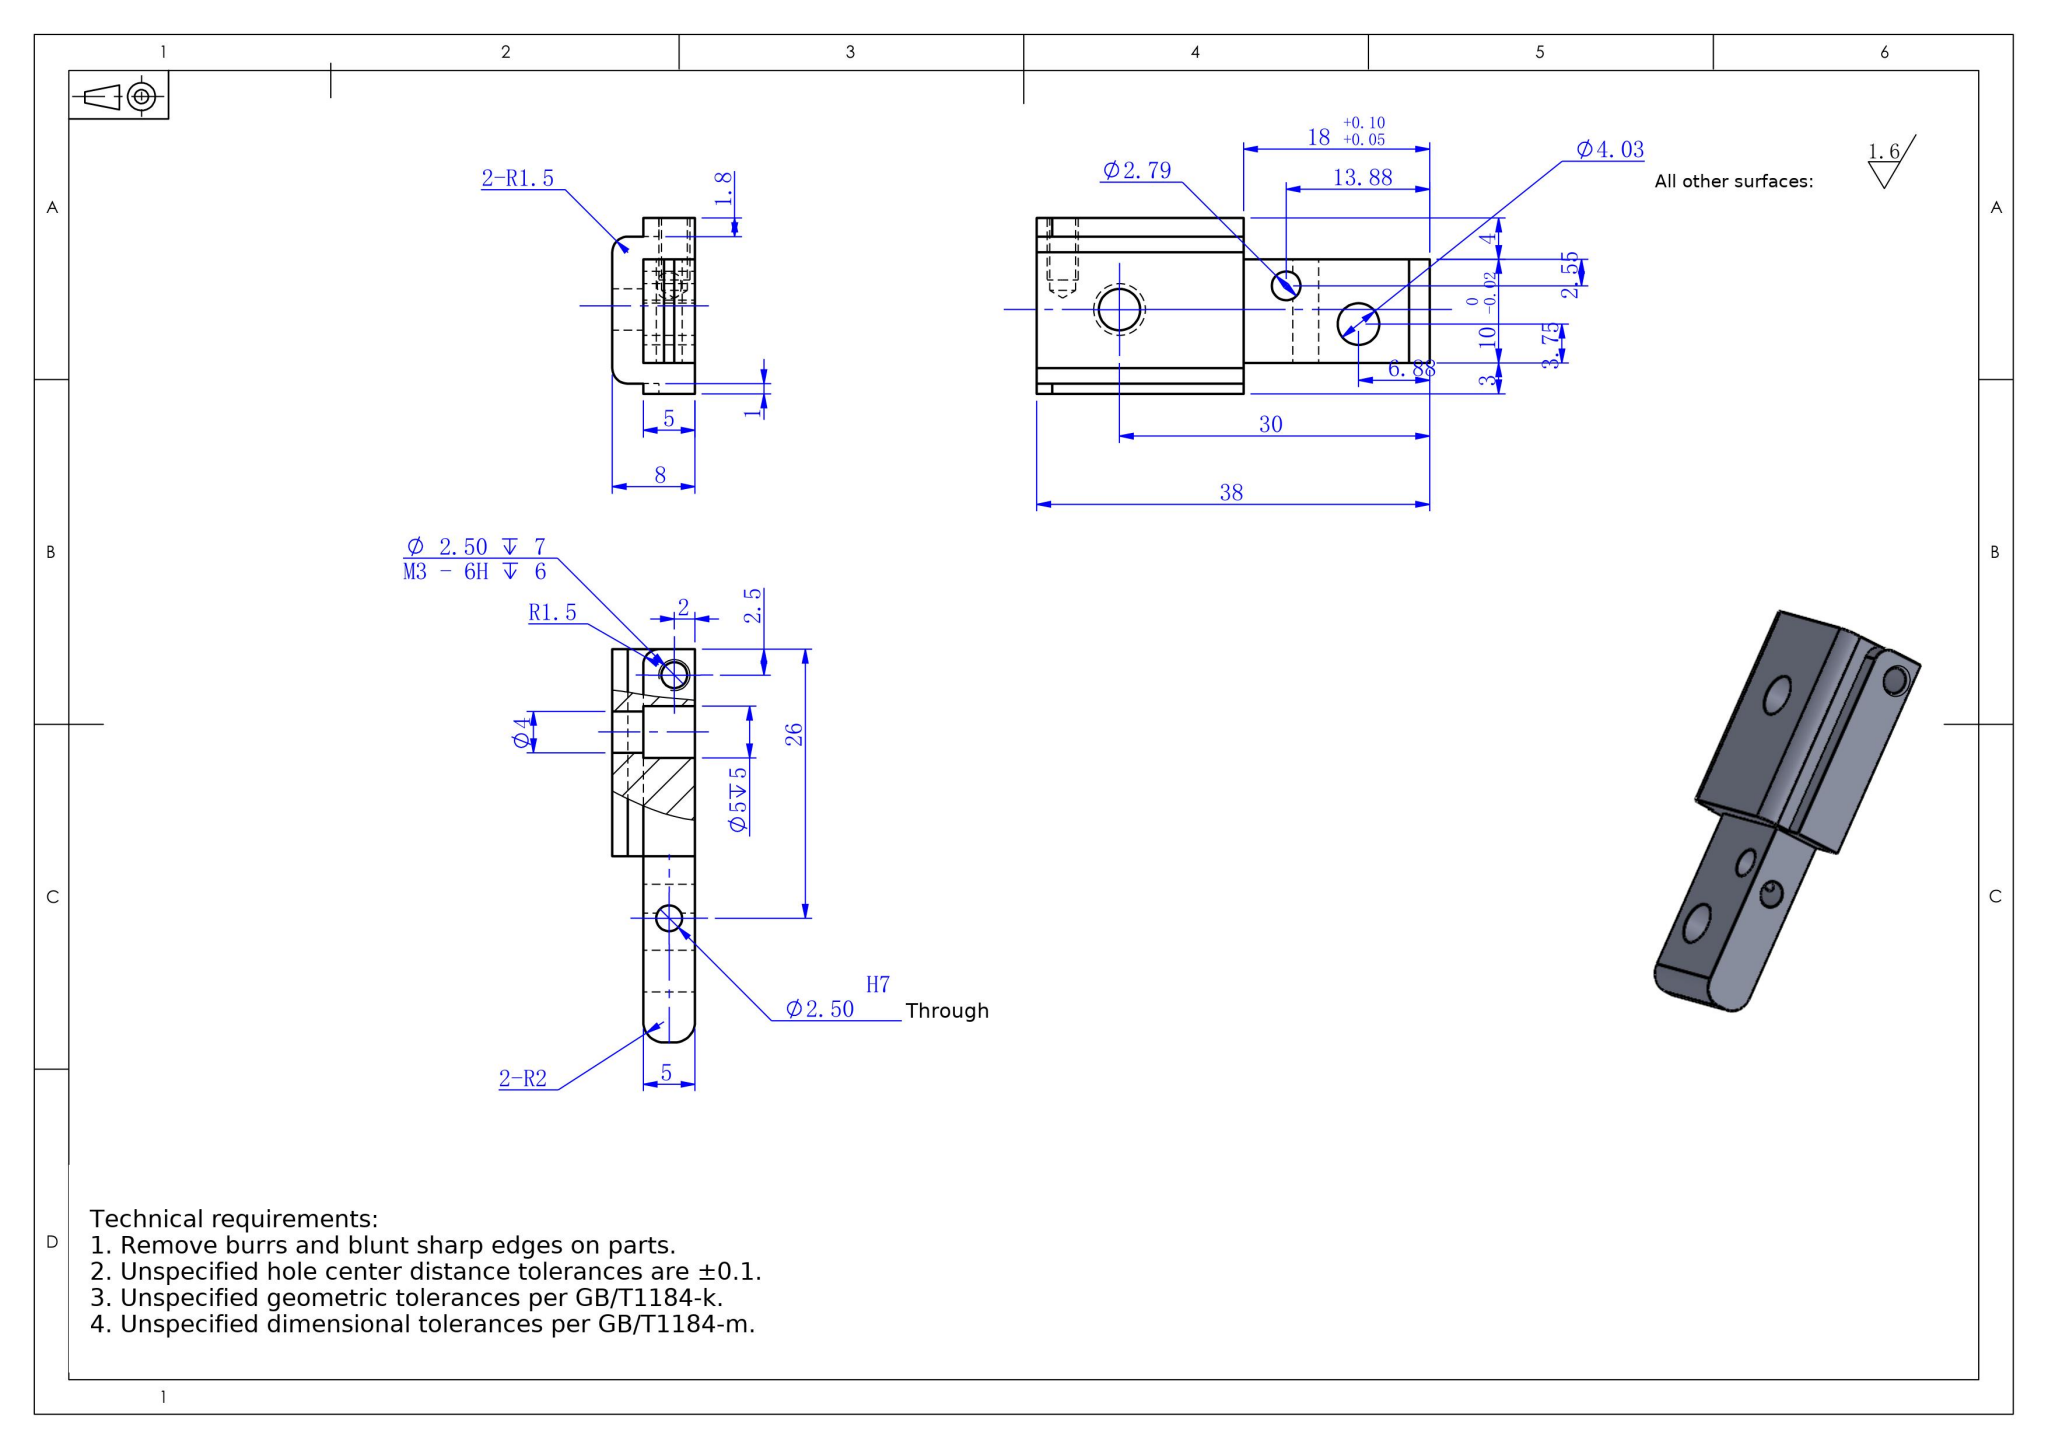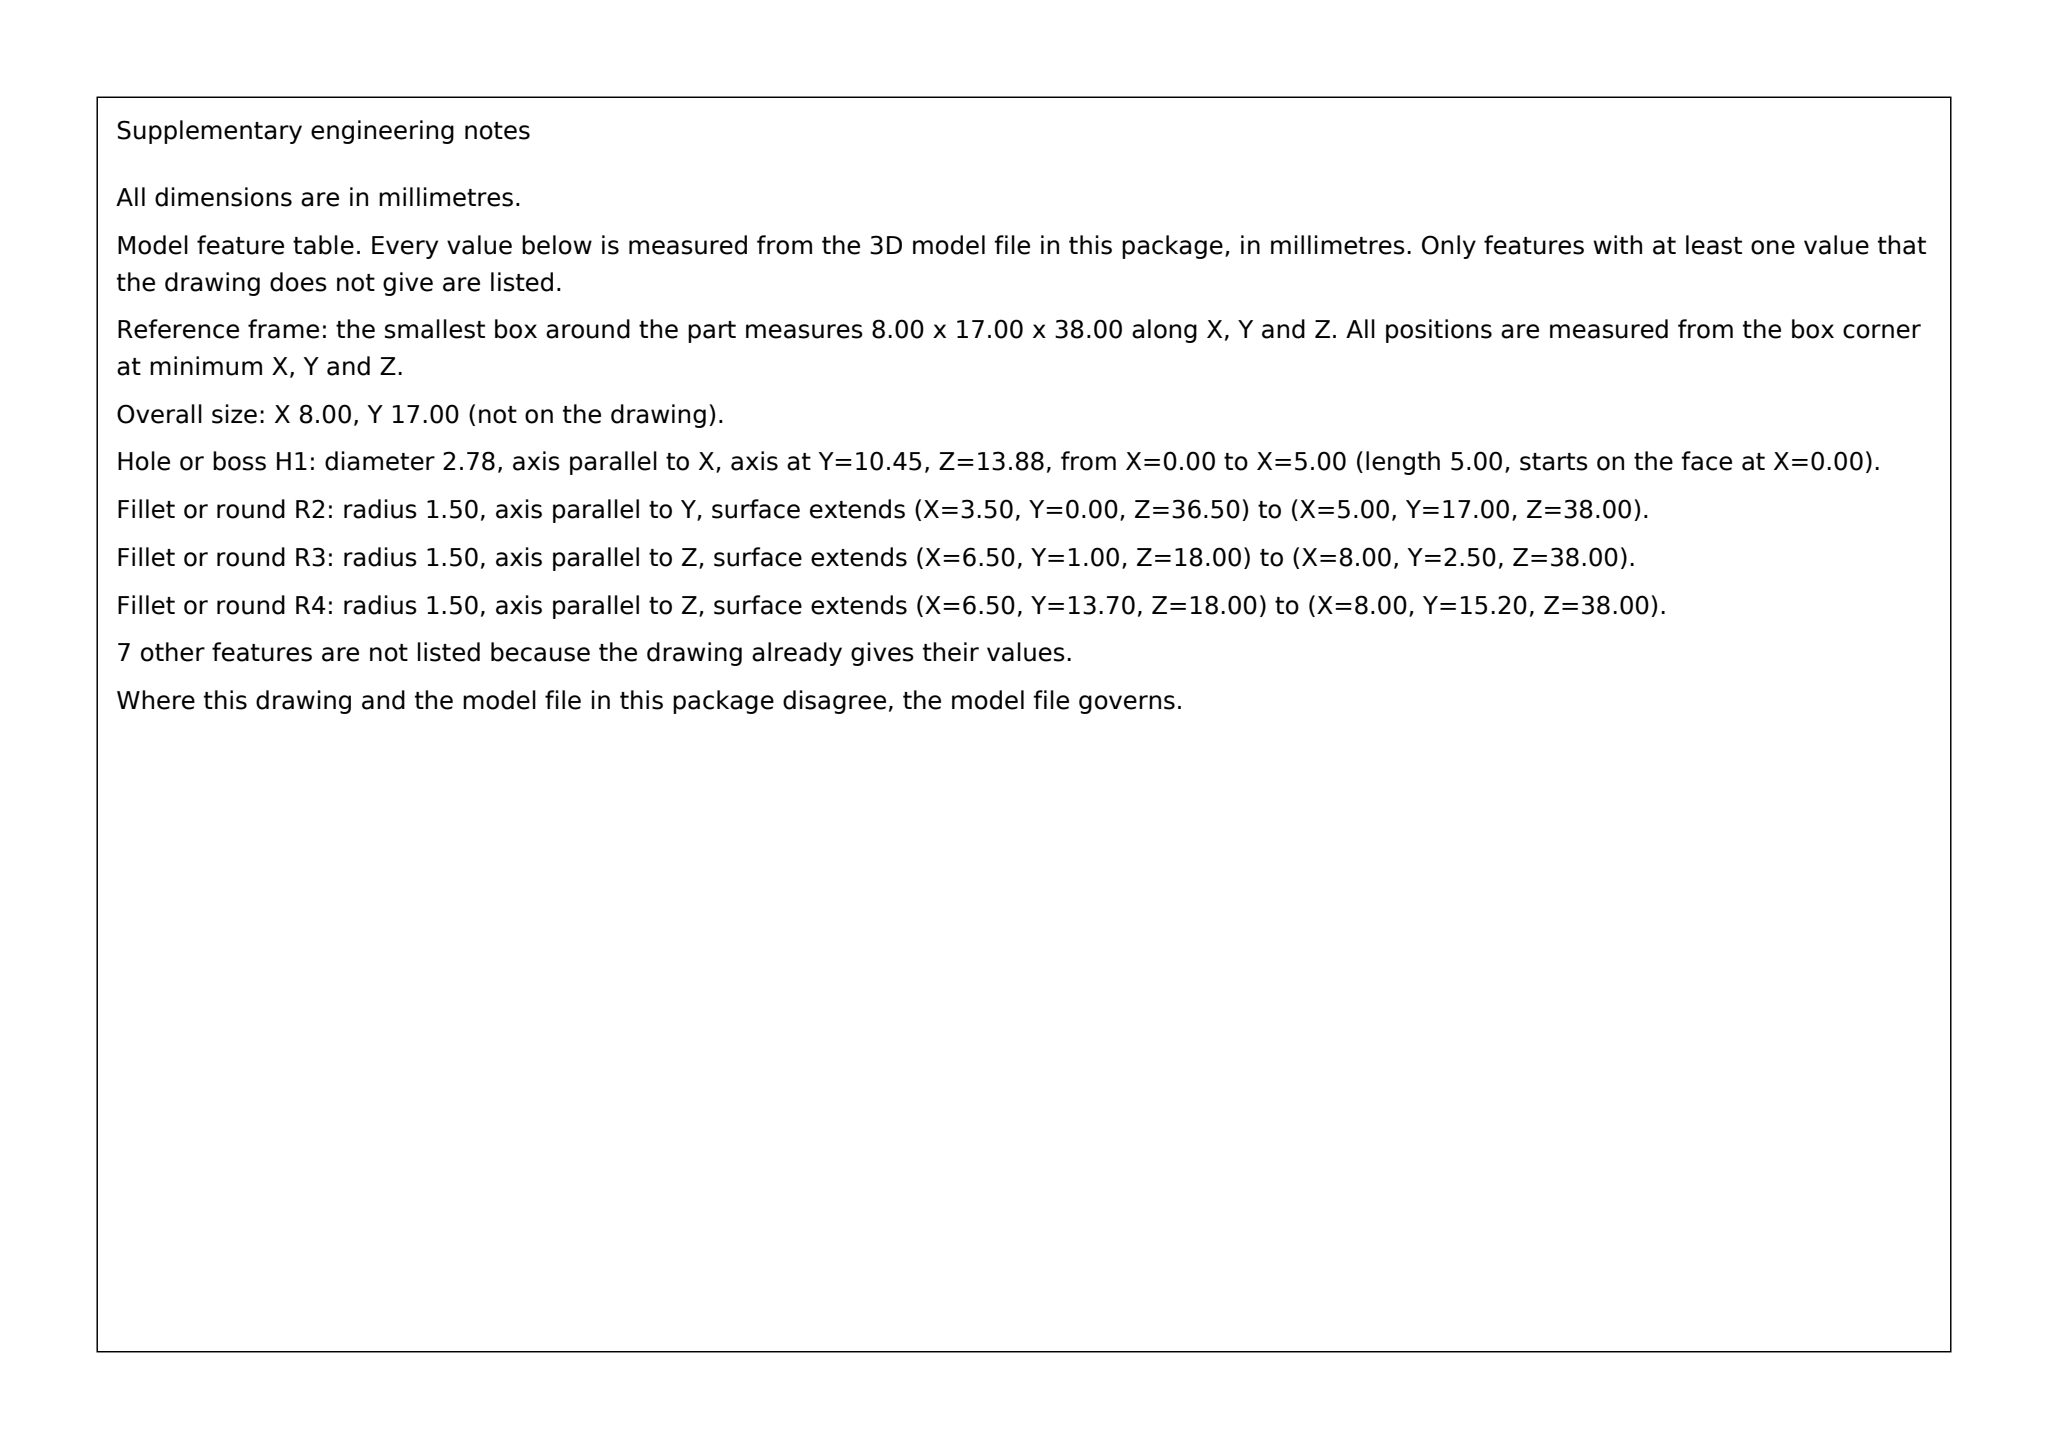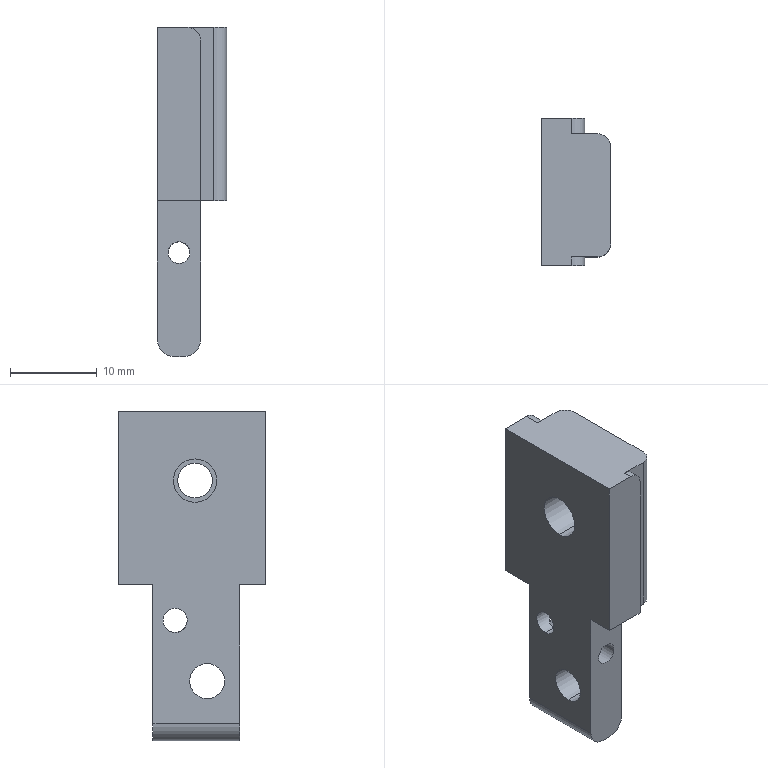Part | SolidWorks | mm | 1 solid | 35 faces | box 8 x 17 x 38 mm | volume 3101 mm3 | cylinder 18 | plane 15 | cone 2 | commonest cylinder face diameters 4 x4 2.5 x4 3 x4 4.029 x2 2.79 x2 5 x2
build123d program:
from build123d import *

# Parameters (mm, degrees)
SKETCH1_W             = 5
SKETCH1_H             = 17
BOSS_EXTRUDE1_DEPTH   = 20
SKETCH2_W             = 5
SKETCH2_H             = 10
BOSS_EXTRUDE2_DEPTH   = 18
SKETCH3_R             = 1.25
CUT_EXTRUDE1_DEPTH    = 55.281
FILLET1_R             = 2
M3_TAPPED_HOLE2_D     = 2.5
M3_TAPPED_HOLE2_DEPTH = 7
M3_TAPPED_HOLE2_TIP   = 0.7511
SKETCH11_W            = 3
SKETCH11_H            = 14.2
BOSS_EXTRUDE3_DEPTH   = 20
SKETCH12_R            = 2.5
CUT_EXTRUDE2_DEPTH    = 5
SKETCH13_R            = 2
CUT_EXTRUDE3_DEPTH    = 10
FILLET2_R             = 1.5
FILLET3_R             = 1.5
SKETCH14_R            = 1.395
SKETCH14_R_2          = 2.015
CUT_EXTRUDE4_DEPTH    = 10


with BuildPart() as part:
    # Sketch1 → Boss-Extrude1 (new body)
    with BuildSketch(Plane.XY):
        with Locations((-46.259, -21.418)):
            Rectangle(SKETCH1_W, SKETCH1_H)
    extrude(amount=BOSS_EXTRUDE1_DEPTH)

    # Sketch2 → Boss-Extrude2 (add)
    with BuildSketch(Plane(origin=(0, 0, 0), x_dir=(-1, 0, 0), z_dir=(0, 0, -1))):
        with Locations((46.259, -21.918)):
            Rectangle(SKETCH2_W, SKETCH2_H)
    extrude(amount=BOSS_EXTRUDE2_DEPTH)

    # Sketch3 → Cut-Extrude1 (cut, through all)
    with BuildSketch(Plane(origin=(0, -16.918, 0), x_dir=(1, 0, 0), z_dir=(0, 1, 0))):
        with Locations(Location((-46.259, 6, 0), (0, 0, 180))):
            Circle(SKETCH3_R)
    extrude(amount=-CUT_EXTRUDE1_DEPTH, mode=Mode.SUBTRACT)

    # Fillet1
    fillet1_edges = [part.edges().sort_by_distance(p)[0] for p in [
        (-43.759, -21.918, -18),
        (-48.759, -21.918, -18),
    ]]
    fillet(fillet1_edges, radius=FILLET1_R)

    # M3 Tapped Hole2
    with Locations(Plane(origin=(0, -12.918, 0), x_dir=(1, 0, 0), z_dir=(0, 1, 0))):
        with Locations((-46.759, -17.5)):
            Hole(M3_TAPPED_HOLE2_D / 2, depth=M3_TAPPED_HOLE2_DEPTH)
            with Locations((0, 0, -(M3_TAPPED_HOLE2_DEPTH + M3_TAPPED_HOLE2_TIP / 2))):  # 118° drill point
                Cone(0, M3_TAPPED_HOLE2_D / 2, M3_TAPPED_HOLE2_TIP, mode=Mode.SUBTRACT)

    # Sketch11 → Boss-Extrude3 (add)
    with BuildSketch(Plane.XY.offset(20)):
        with Locations((-42.259, -21.818)):
            Rectangle(SKETCH11_W, SKETCH11_H)
    extrude(amount=-BOSS_EXTRUDE3_DEPTH)

    # Sketch12 → Cut-Extrude2 (cut)
    with BuildSketch(Plane.ZY.offset(48.759)):
        with Locations((12, -21.768)):
            Circle(SKETCH12_R)
    extrude(amount=-CUT_EXTRUDE2_DEPTH, mode=Mode.SUBTRACT)

    # Sketch13 → Cut-Extrude3 (cut)
    with BuildSketch(Plane.ZY.offset(43.759)):
        with Locations((12, -21.768)):
            Circle(SKETCH13_R)
    extrude(amount=-CUT_EXTRUDE3_DEPTH, mode=Mode.SUBTRACT)

    # Fillet2
    fillet2_edges = [part.edges().sort_by_distance(p)[0] for p in [
        (-40.759, -14.718, 10),
        (-40.759, -28.918, 10),
    ]]
    fillet(fillet2_edges, radius=FILLET2_R)

    # Fillet3
    fillet3_edges = [part.edges().sort_by_distance(p)[0] for p in [
        (-43.759, -29.418, 20),
        (-43.759, -13.818, 20),
    ]]
    fillet(fillet3_edges, radius=FILLET3_R)

    # Sketch14 → Cut-Extrude4 (cut)
    with BuildSketch(Plane(origin=(-43.759, 0, 0), x_dir=(0, 0, -1), z_dir=(1, 0, 0))):
        with Locations((4.119, -19.47)):
            Circle(SKETCH14_R)
        with Locations((11.116, -23.167)):
            Circle(SKETCH14_R_2)
    extrude(amount=-CUT_EXTRUDE4_DEPTH, mode=Mode.SUBTRACT)


solid = part.part